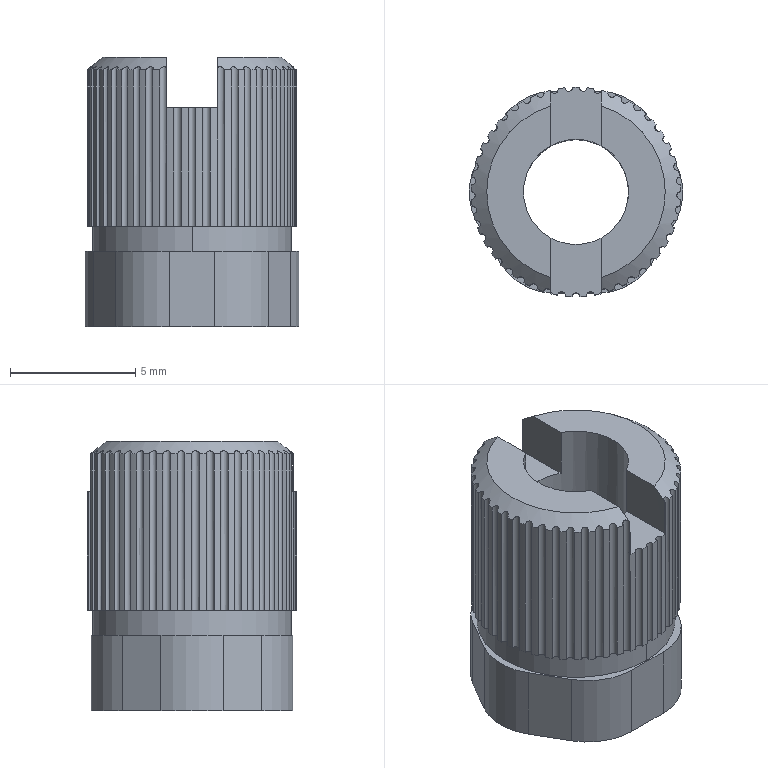CAM job | Mastercam | mm | 10 operations | part box 8.54 x 8.37 x 10.75
1. Contour (Ramp) | 2 - 4 平铣刀
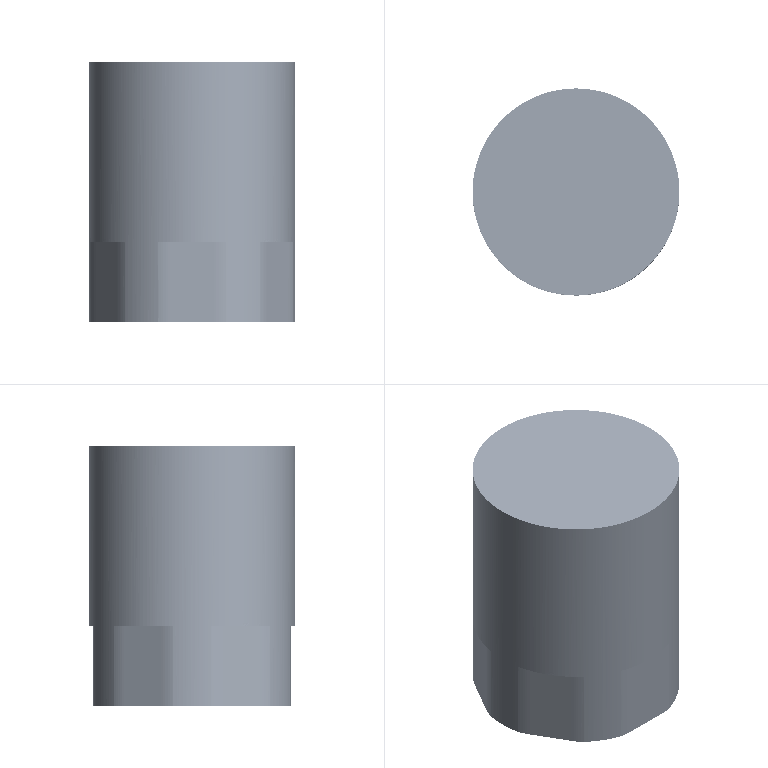2. Contour (2D) | 2 - 4 平铣刀
3. Contour (2D chamfer) | 7 - 4 倒角刀
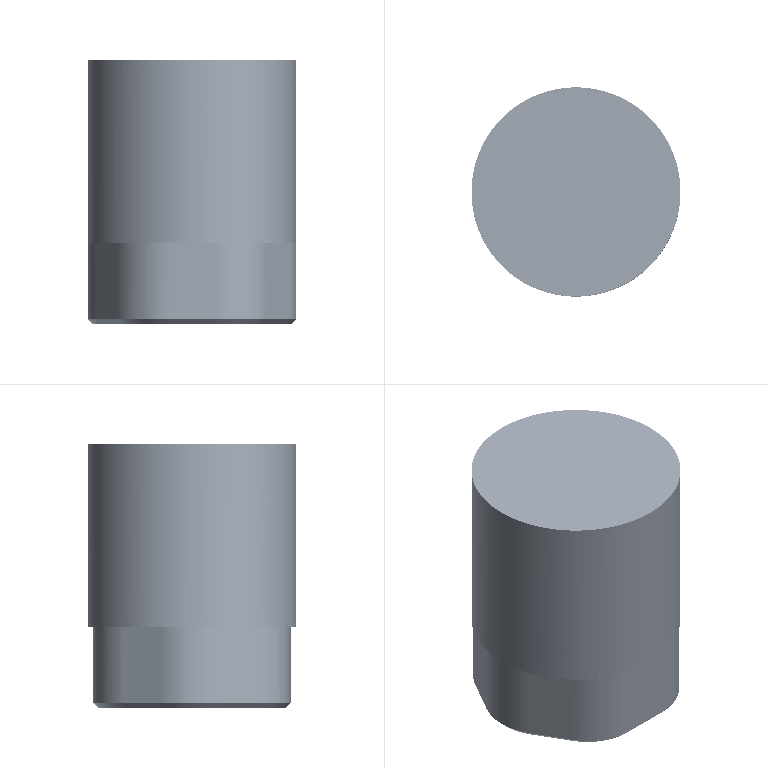4. Contour (Ramp) | 4 - 4 平铣刀
5. Contour (Ramp) | 4 - 4 平铣刀
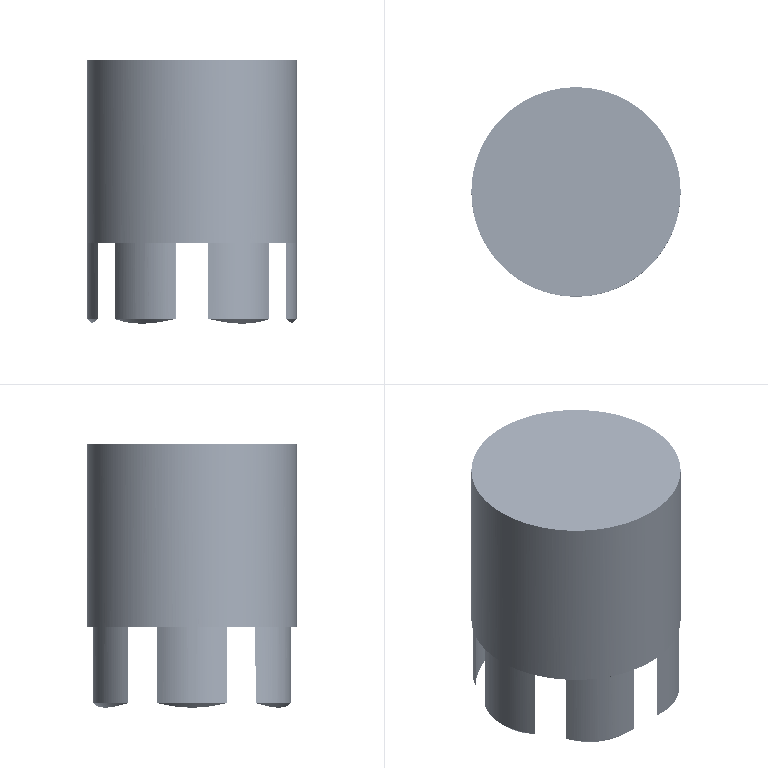6. Contour (Ramp) | 4 - 4 平铣刀
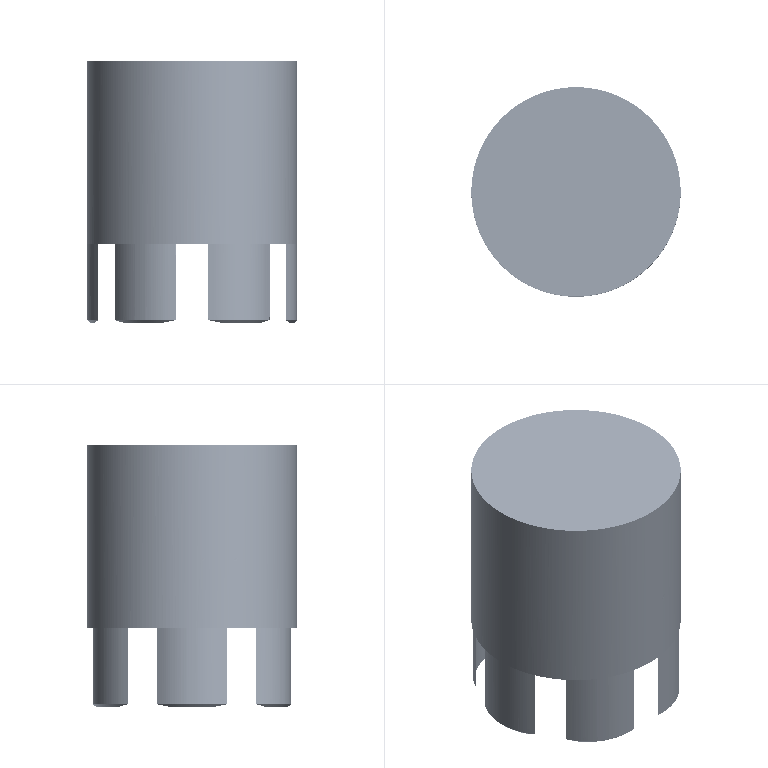7. Contour (Ramp) | 4 - 4 平铣刀
8. Contour (Ramp) | 2 - 2 平铣刀
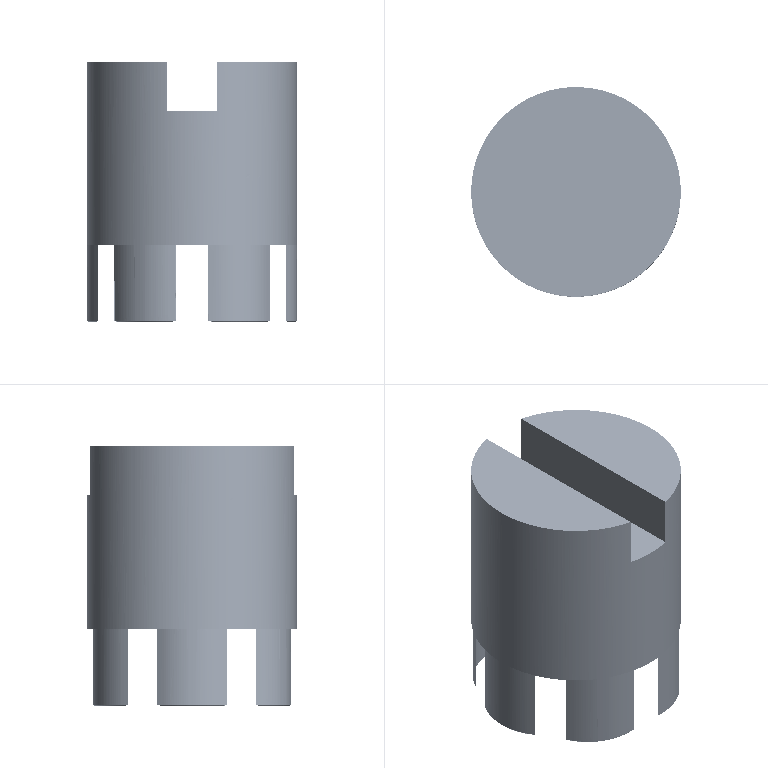9. Contour (2D) | 2 - 2 平铣刀
10. Contour (2D chamfer) | 7 - 4 倒角刀